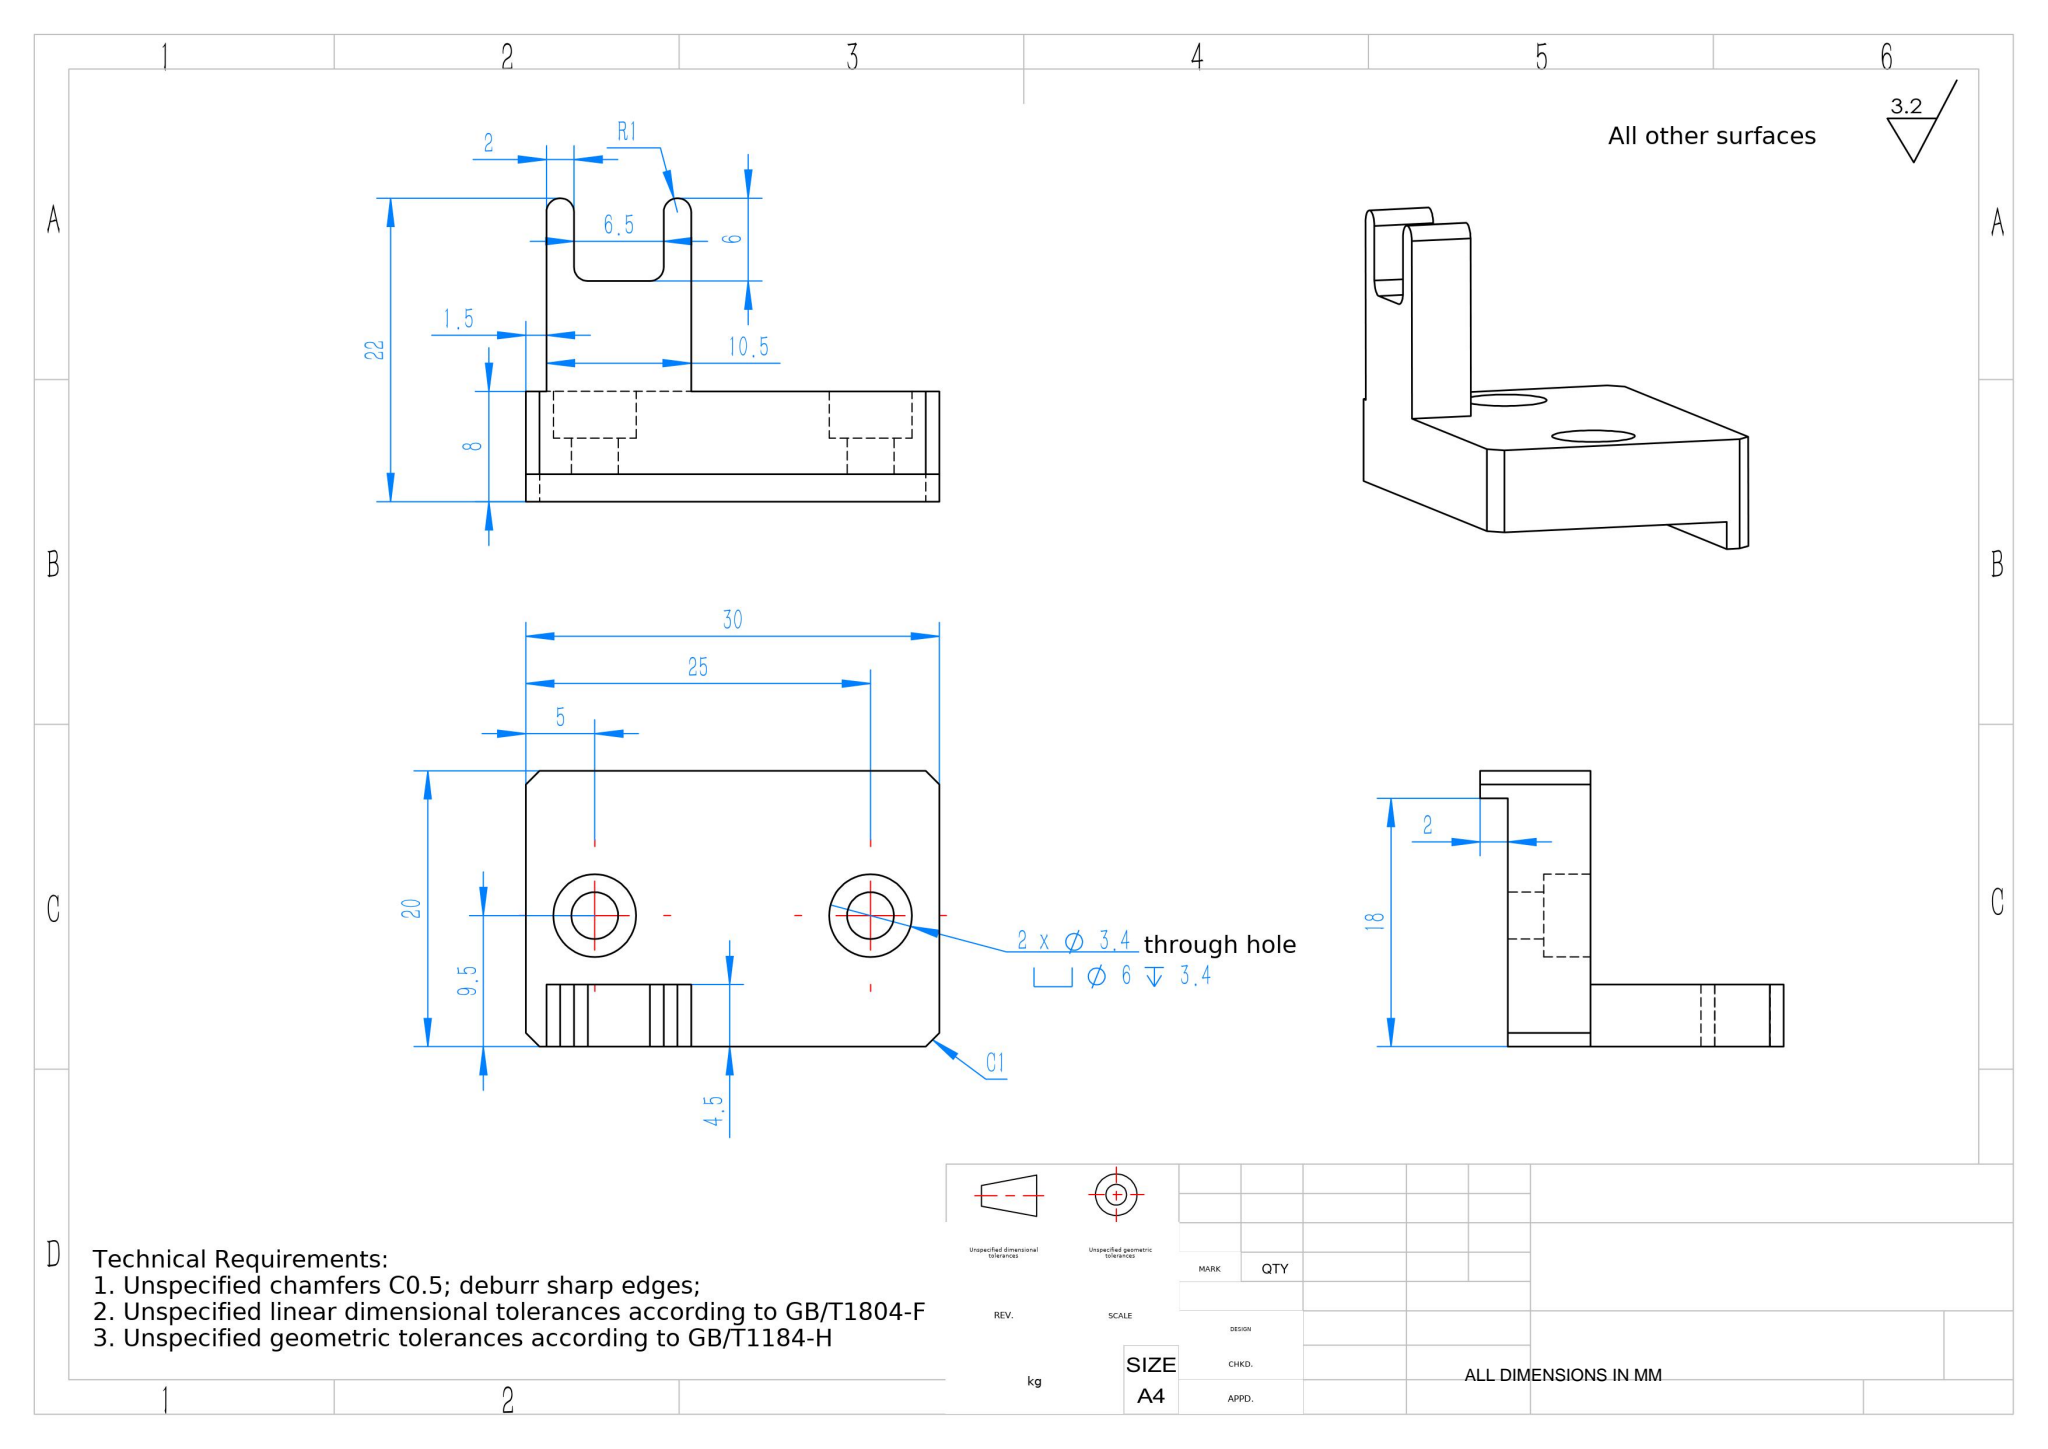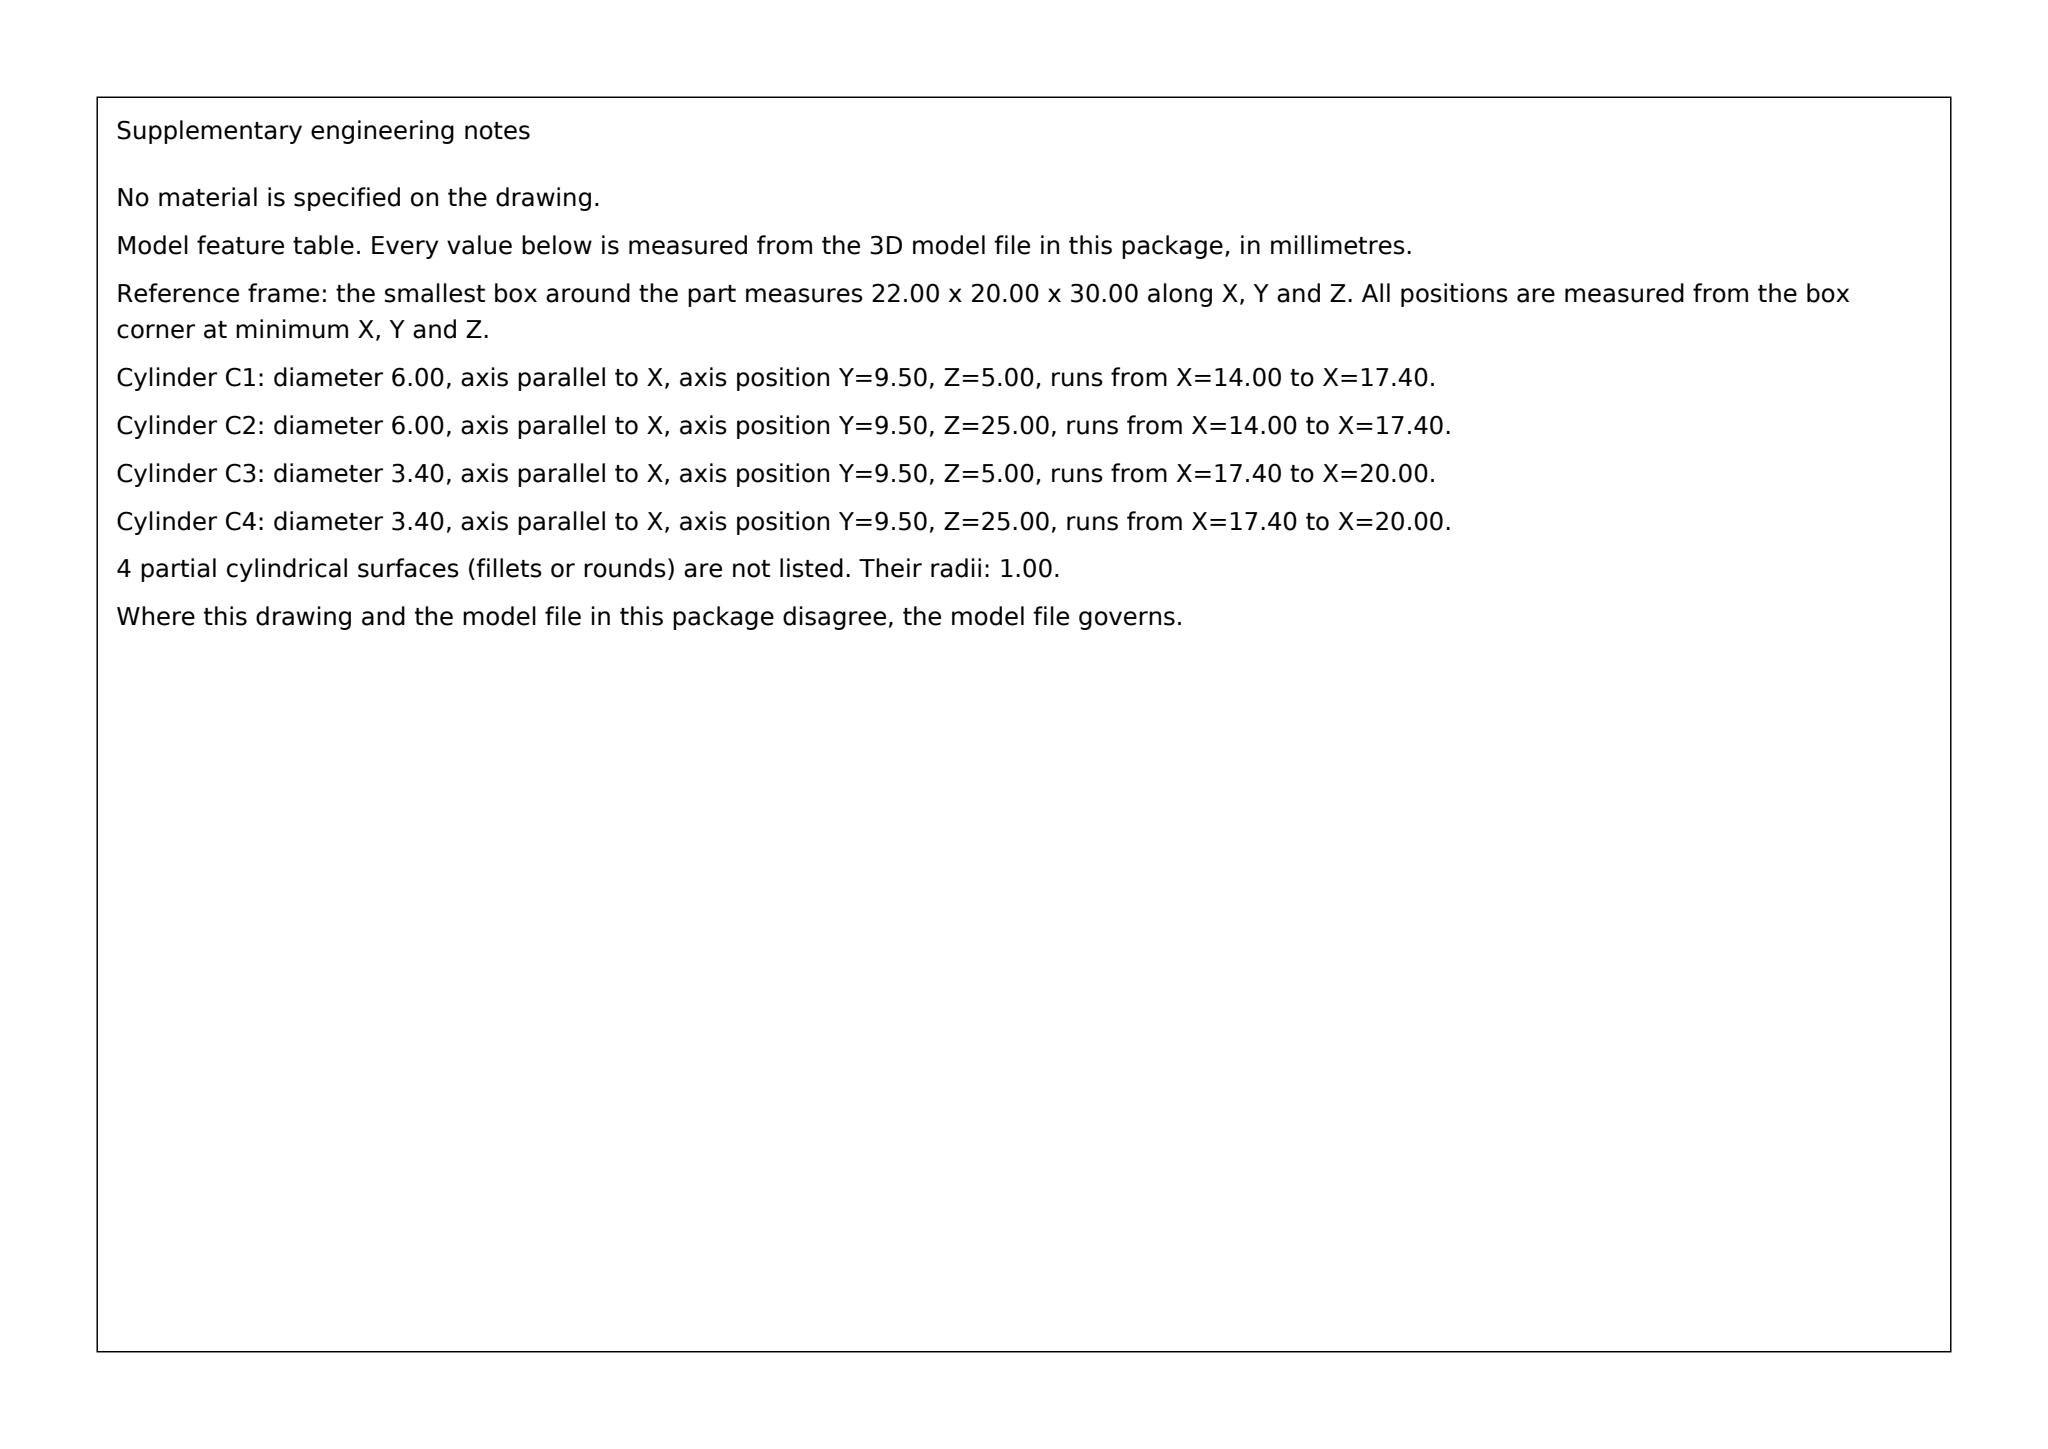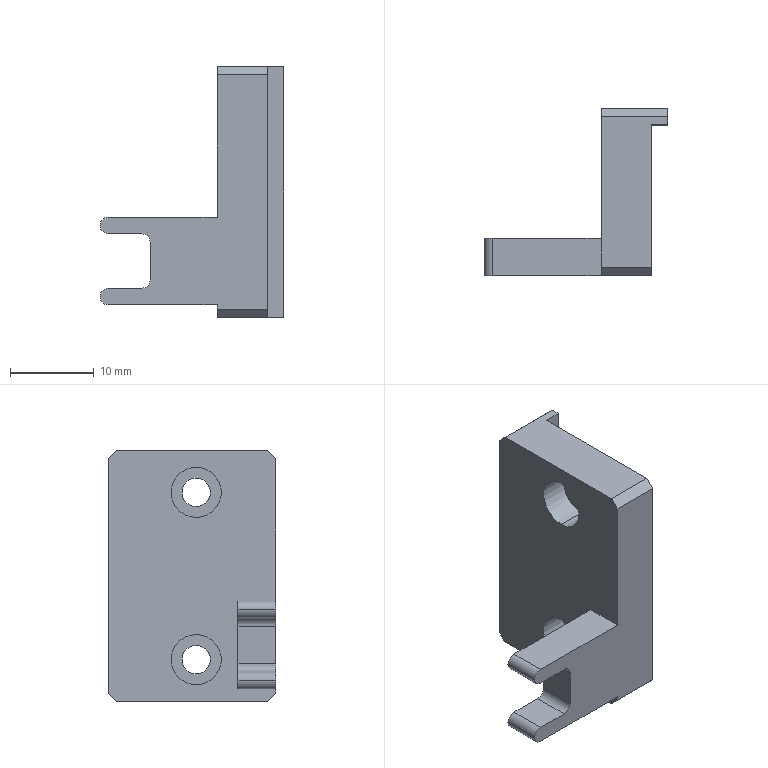Part | SolidWorks | mm | 1 solid | 34 faces | box 22 x 20 x 30 mm | volume 3951 mm3 | plane 20 | cylinder 14 | commonest cylinder face diameters 2 x6 6 x4 3.4 x4